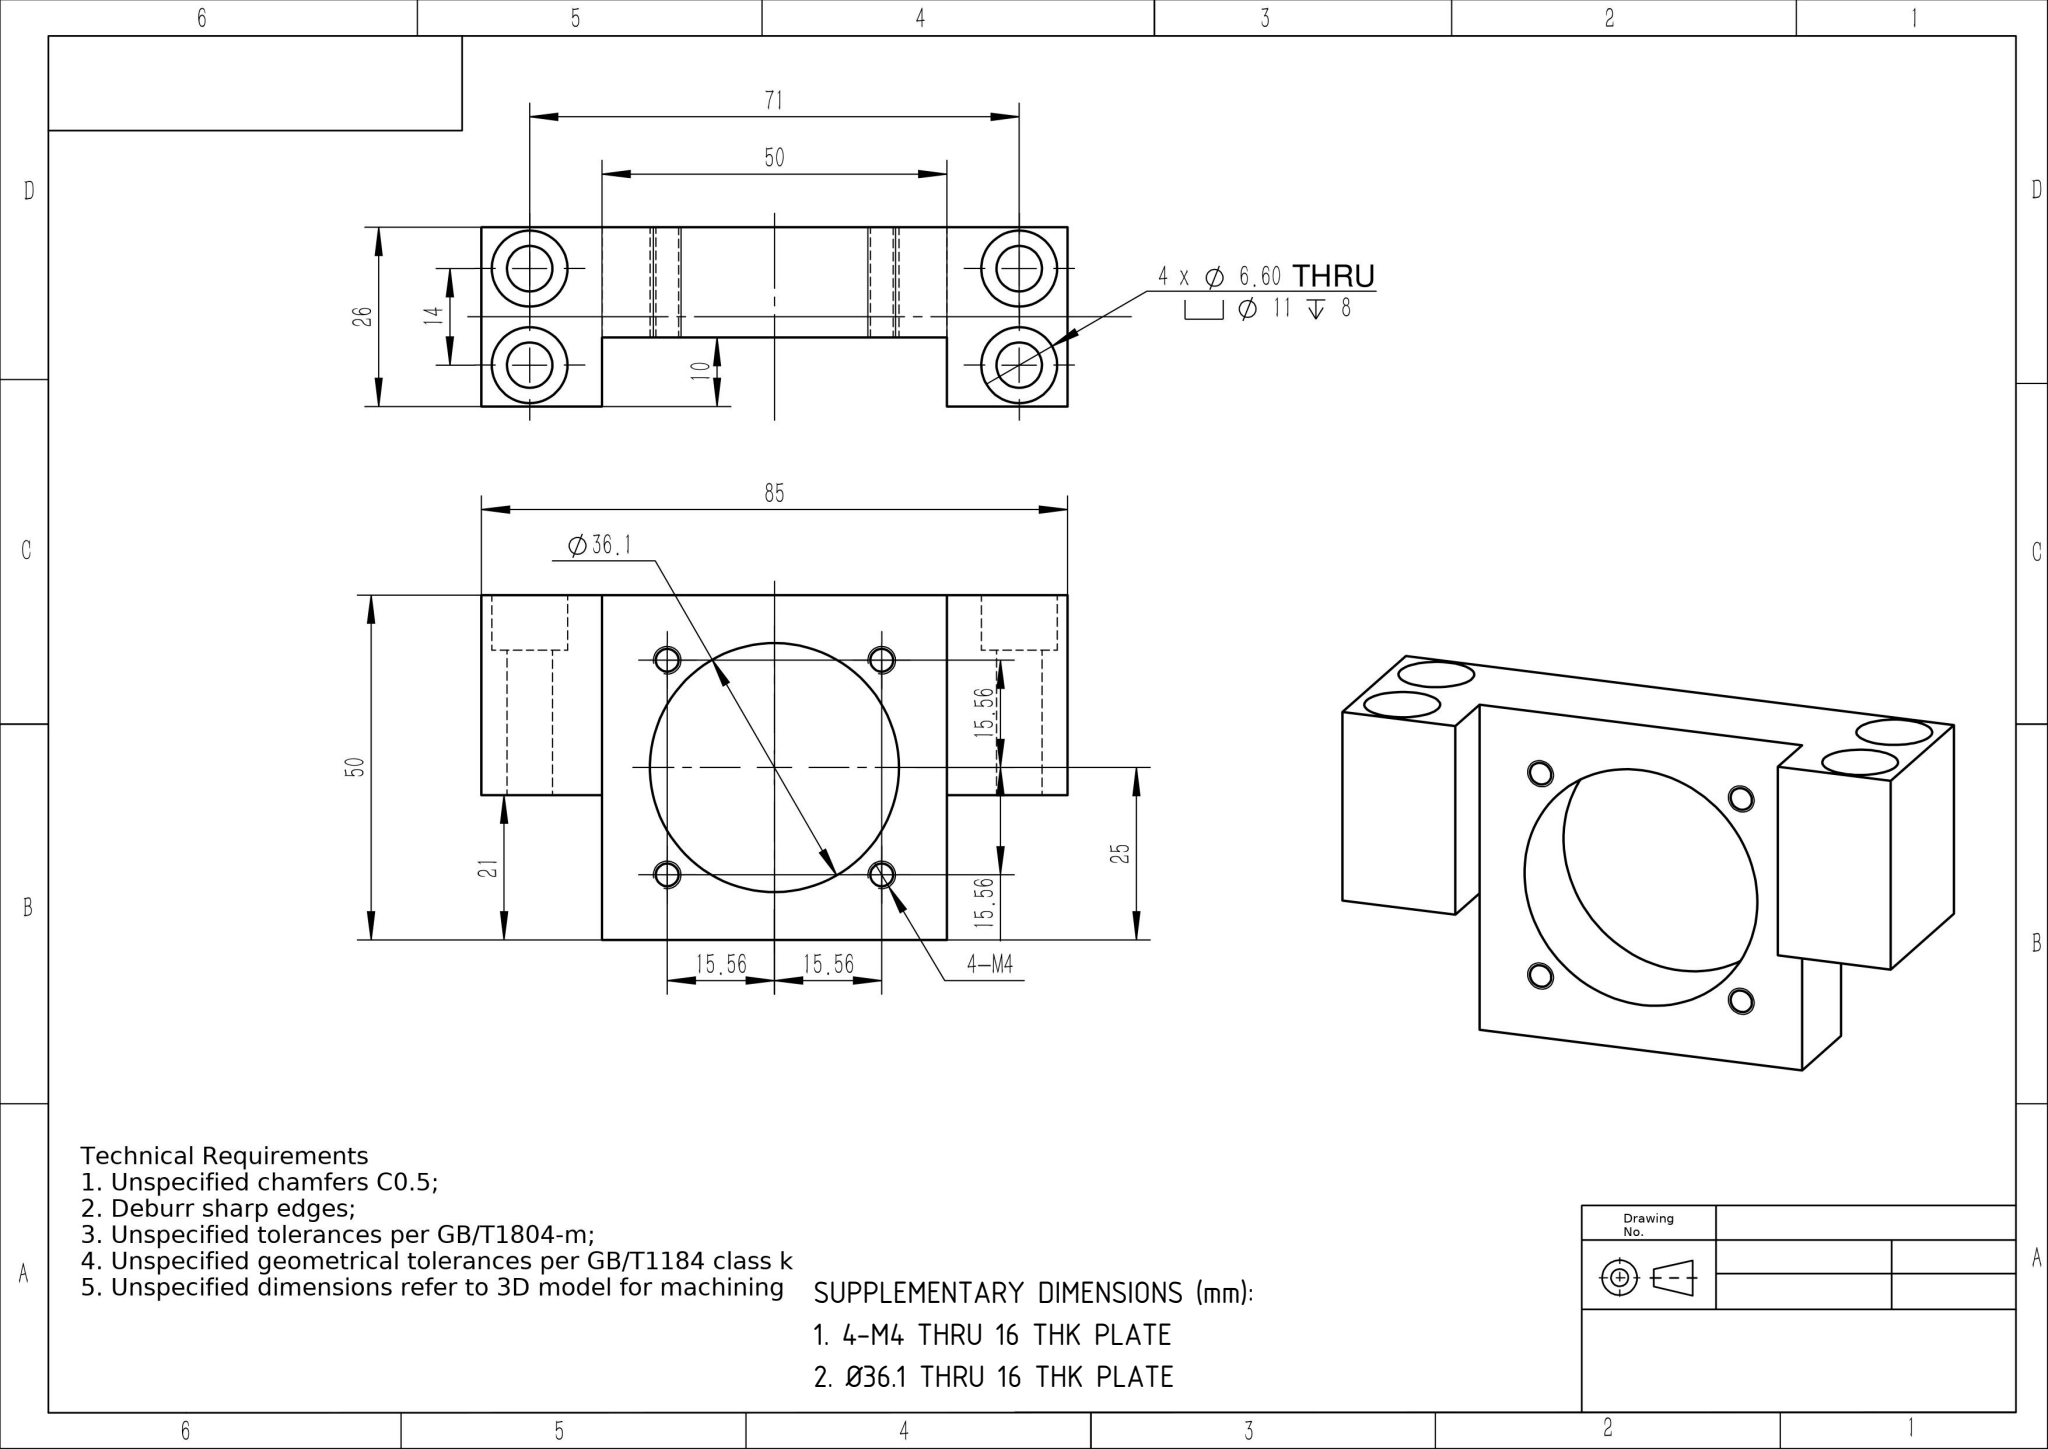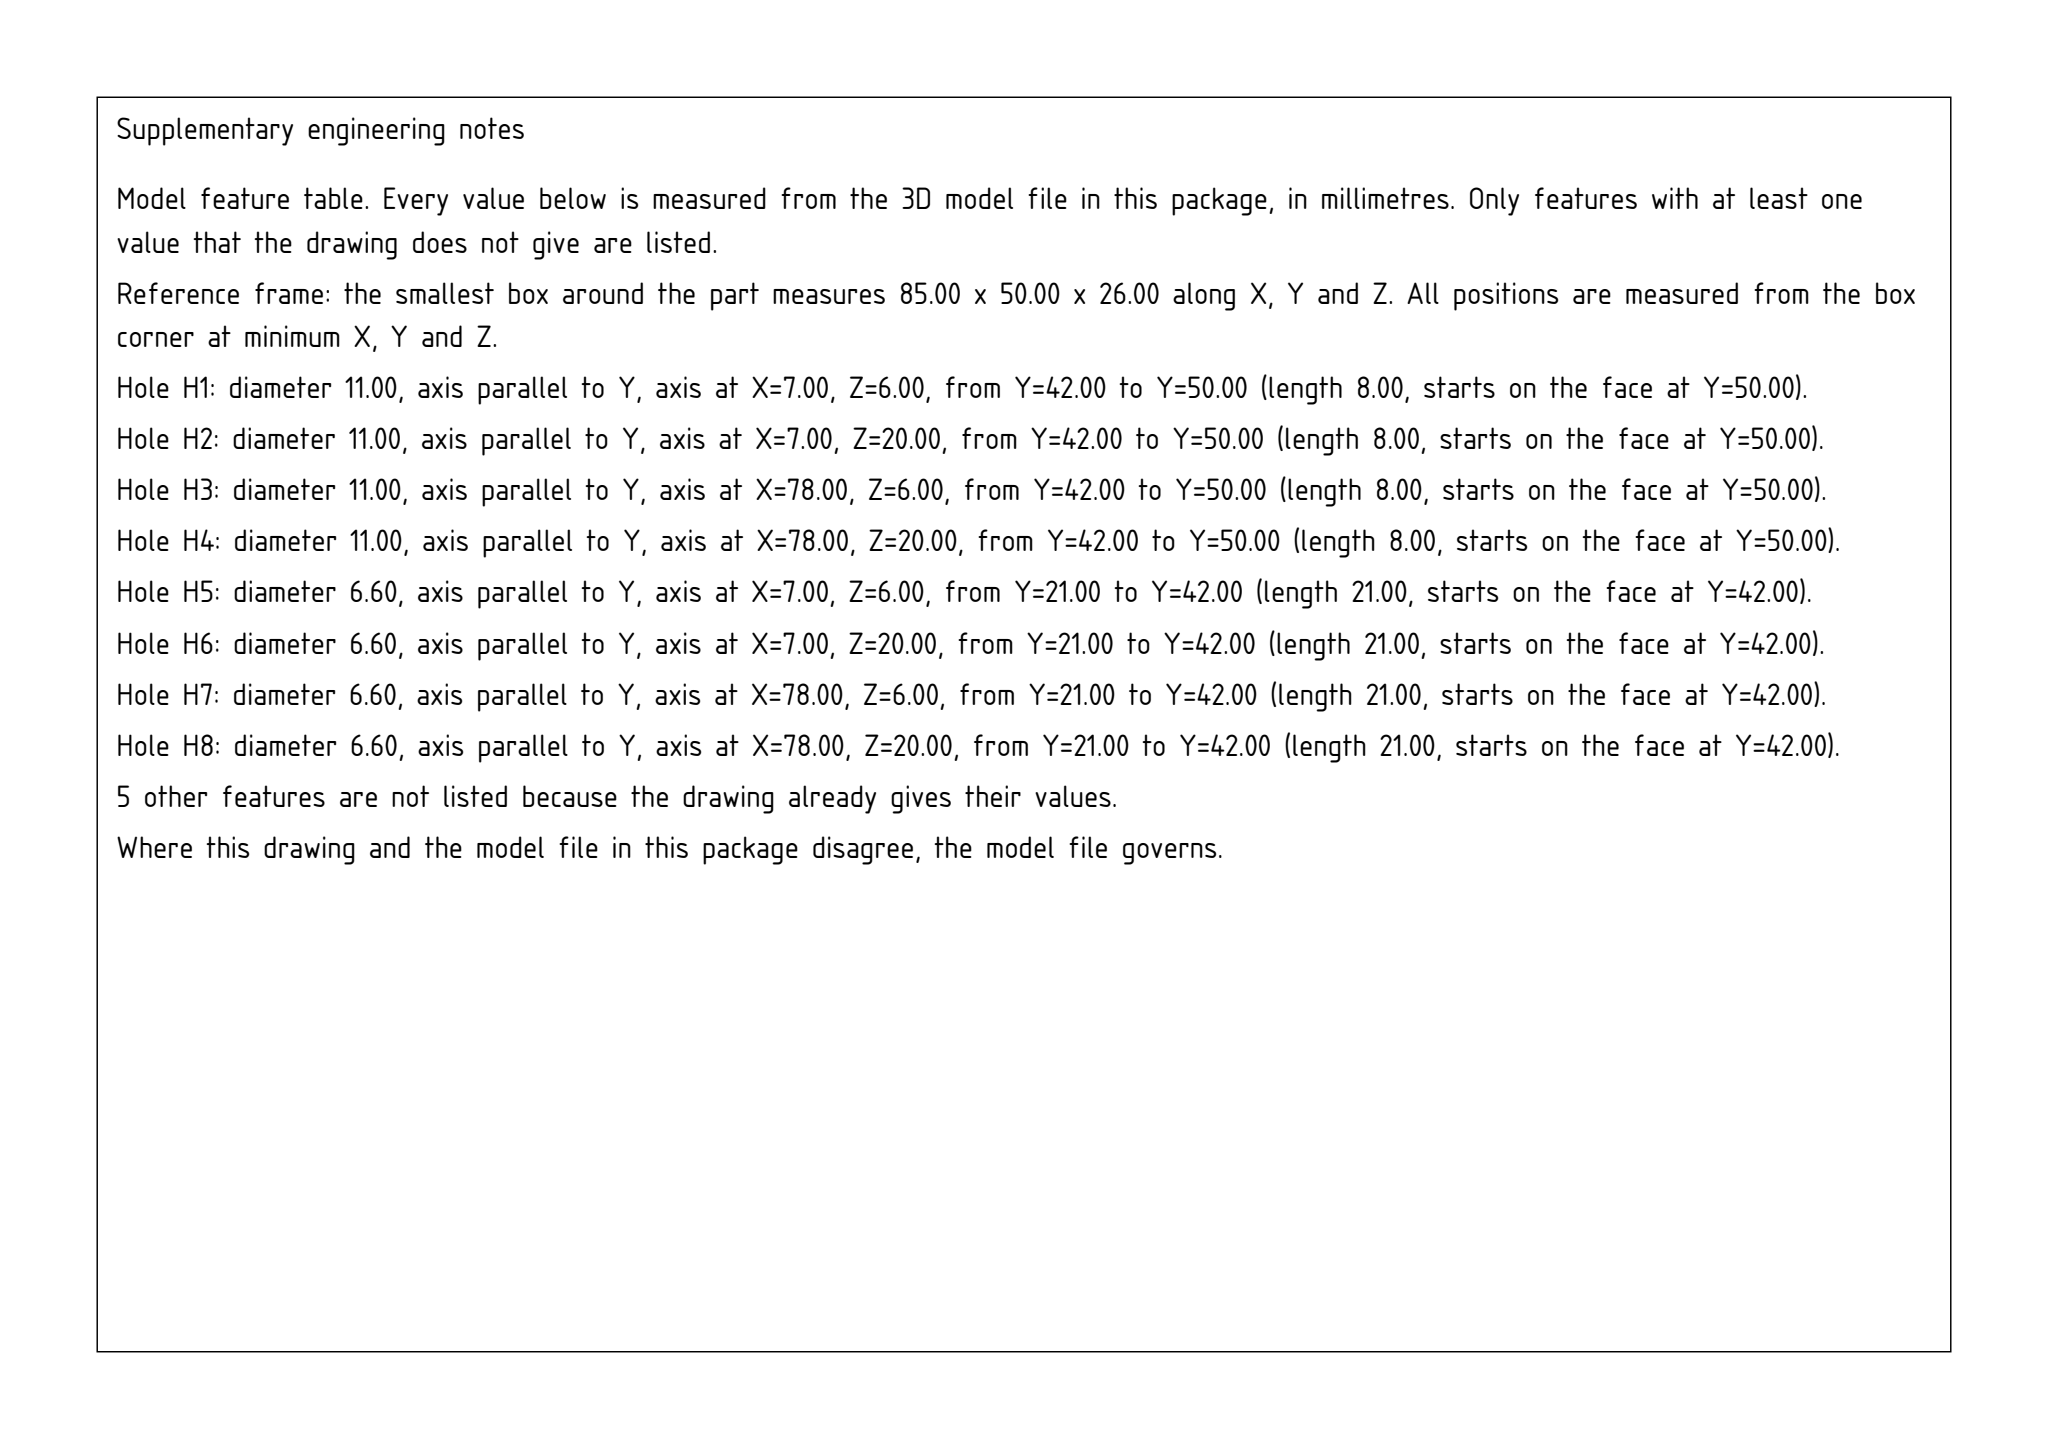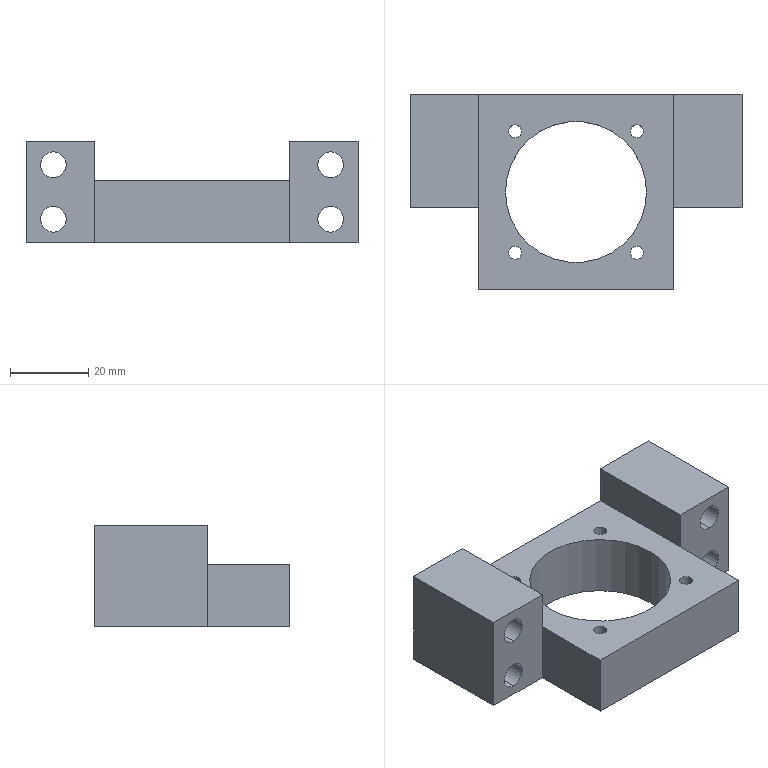Part | SolidWorks | mm | 1 solid | 44 faces | box 85 x 50 x 26 mm | volume 43551 mm3 | cylinder 26 | plane 18 | commonest cylinder face diameters 3.3 x8 11 x8 6.6 x8 36.1 x2
build123d program:
from build123d import *

# Parameters (mm, degrees)
SKETCH1_W                                            = 85
SKETCH1_H                                            = 50
BOSS_EXTRUDE1_DEPTH                                  = 13
SKETCH2_W                                            = 50
SKETCH2_H                                            = 50
CUT_EXTRUDE1_DEPTH                                   = 10
SKETCH3_W                                            = 17.5
SKETCH3_H                                            = 21
CUT_EXTRUDE2_DEPTH                                   = 56.743
SKETCH4_R                                            = 18.05
CUT_EXTRUDE3_DEPTH                                   = 52.839
HOLE_SIZE_ACCORDING_TO_TYPE_1_OF_HEXAGON_D           = 6.6
HOLE_SIZE_ACCORDING_TO_TYPE_1_OF_HEXAGON_CBORE_D     = 11
HOLE_SIZE_ACCORDING_TO_TYPE_1_OF_HEXAGON_CBORE_DEPTH = 8
M4_TAPPED_HOLE1_D                                    = 3.3


with BuildPart() as part:
    # Sketch1 → Boss-Extrude1 (new, symmetric)
    with BuildSketch(Plane.XY):
        Rectangle(SKETCH1_W, SKETCH1_H)
    extrude(amount=BOSS_EXTRUDE1_DEPTH, both=True)

    # Sketch2 → Cut-Extrude1 (cut)
    with BuildSketch(Plane.XY.offset(13)):
        Rectangle(SKETCH2_W, SKETCH2_H)
    extrude(amount=-CUT_EXTRUDE1_DEPTH, mode=Mode.SUBTRACT)

    # Sketch3 → Cut-Extrude2 (cut, through all)
    with BuildSketch(Plane.XY.offset(13)):
        with Locations((-33.75, -14.5)):
            Rectangle(SKETCH3_W, SKETCH3_H)
        with Locations((33.75, -14.5)):
            Rectangle(SKETCH3_W, SKETCH3_H)
    extrude(amount=-CUT_EXTRUDE2_DEPTH, mode=Mode.SUBTRACT)

    # Sketch4 → Cut-Extrude3 (cut, through all)
    with BuildSketch(Plane.XY.offset(3)):
        Circle(SKETCH4_R)
    extrude(amount=-CUT_EXTRUDE3_DEPTH, mode=Mode.SUBTRACT)

    # Hole Size_According to_Type 1 of Hexagon (through all)
    with Locations(Plane(origin=(0, 25, 0), x_dir=(1, 0, 0), z_dir=(0, 1, 0))):
        with Locations((-35.5, 7), (-35.5, -7), (35.5, 7), (35.5, -7)):
            CounterBoreHole(HOLE_SIZE_ACCORDING_TO_TYPE_1_OF_HEXAGON_D / 2, HOLE_SIZE_ACCORDING_TO_TYPE_1_OF_HEXAGON_CBORE_D / 2, HOLE_SIZE_ACCORDING_TO_TYPE_1_OF_HEXAGON_CBORE_DEPTH)

    # M4 Tapped Hole1 (through all)
    with Locations(Plane.XY.offset(3)):
        with Locations((-15.556, 15.556), (15.556, 15.556), (-15.556, -15.556), (15.556, -15.556)):
            Hole(M4_TAPPED_HOLE1_D / 2)


solid = part.part